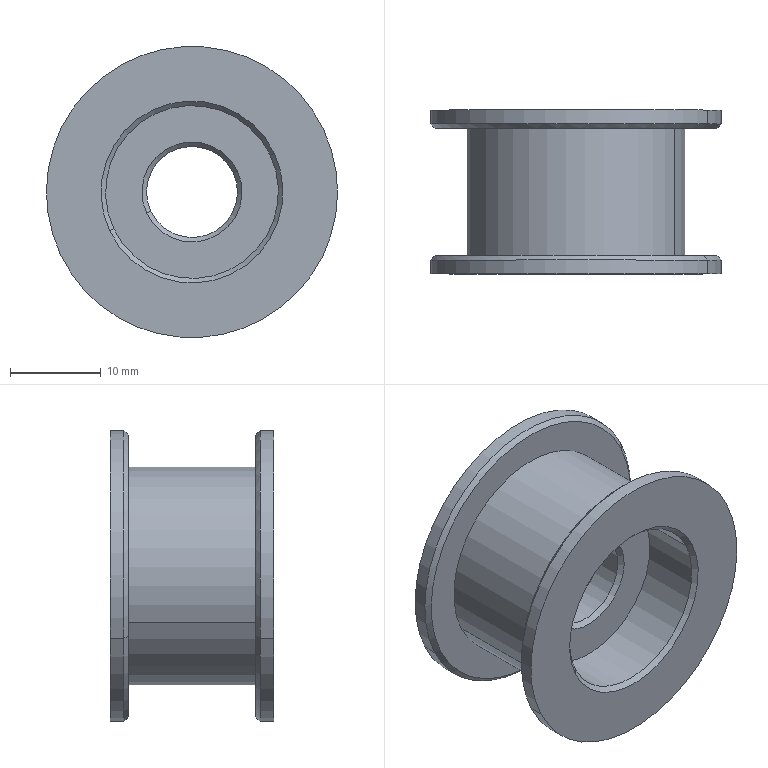Component | SolidWorks | Roller-1_BearingSleeve-1 | 1 solid | 30 faces | box 32 x 18 x 32 mm | volume 5219 mm3 | cone 12 | cylinder 12 | plane 6 | commonest cylinder face diameters 32 x4 19 x4 10 x2 24 x2
STEP:
#1=CARTESIAN_POINT('',(2.401,-2.146,10.487));
#2=VERTEX_POINT('',#1);
#3=CARTESIAN_POINT('',(3.505,-2.146,11.009));
#4=VERTEX_POINT('',#3);
#5=CARTESIAN_POINT('',(2.953,-2.146,10.748));
#6=DIRECTION('',(0.,1.,0.));
#7=DIRECTION('',(0.9043,0.,0.4269));
#8=AXIS2_PLACEMENT_3D('',#5,#6,#7);
#9=CIRCLE('',#8,0.6102);
#10=EDGE_CURVE('',#2,#4,#9,.T.);
#11=ORIENTED_EDGE('',*,*,#10,.F.);
#12=CARTESIAN_POINT('',(2.383,-2.165,10.479));
#13=VERTEX_POINT('',#12);
#14=CARTESIAN_POINT('',(2.383,-2.165,10.479));
#15=DIRECTION('',(-0.6394,-0.7071,-0.3019));
#16=VECTOR('',#15,39.37);
#17=LINE('',#14,#16);
#18=EDGE_CURVE('',#2,#13,#17,.T.);
#19=ORIENTED_EDGE('',*,*,#18,.T.);
#20=CARTESIAN_POINT('',(3.522,-2.165,11.017));
#21=VERTEX_POINT('',#20);
#22=CARTESIAN_POINT('',(2.953,-2.165,10.748));
#23=DIRECTION('',(0.,-1.,0.));
#24=DIRECTION('',(0.9043,0.,0.4269));
#25=AXIS2_PLACEMENT_3D('',#22,#23,#24);
#26=CIRCLE('',#25,0.6299);
#27=EDGE_CURVE('',#21,#13,#26,.T.);
#28=ORIENTED_EDGE('',*,*,#27,.F.);
#29=CARTESIAN_POINT('',(3.522,-2.165,11.017));
#30=DIRECTION('',(0.6394,-0.7071,0.3019));
#31=VECTOR('',#30,39.37);
#32=LINE('',#29,#31);
#33=EDGE_CURVE('',#4,#21,#32,.T.);
#34=ORIENTED_EDGE('',*,*,#33,.F.);
#35=EDGE_LOOP('',(#11,#19,#28,#34));
#36=FACE_OUTER_BOUND('',#35,.T.);
#37=CARTESIAN_POINT('',(2.953,-2.165,10.748));
#38=DIRECTION('',(0.,-1.,0.));
#39=DIRECTION('',(0.9043,0.,0.4269));
#40=AXIS2_PLACEMENT_3D('',#37,#38,#39);
#41=CONICAL_SURFACE('',#40,0.6299,0.7854);
#42=ADVANCED_FACE('',(#36),#41,.T.);
#43=CARTESIAN_POINT('',(3.505,-1.594,11.009));
#44=VERTEX_POINT('',#43);
#45=CARTESIAN_POINT('',(2.401,-1.594,10.487));
#46=VERTEX_POINT('',#45);
#47=CARTESIAN_POINT('',(2.953,-1.594,10.748));
#48=DIRECTION('',(0.,-1.,0.));
#49=DIRECTION('',(-0.9043,0.,-0.4269));
#50=AXIS2_PLACEMENT_3D('',#47,#48,#49);
#51=CIRCLE('',#50,0.6102);
#52=EDGE_CURVE('',#44,#46,#51,.T.);
#53=ORIENTED_EDGE('',*,*,#52,.F.);
#54=CARTESIAN_POINT('',(3.522,-1.575,11.017));
#55=VERTEX_POINT('',#54);
#56=CARTESIAN_POINT('',(3.522,-1.575,11.017));
#57=DIRECTION('',(0.6394,0.7071,0.3019));
#58=VECTOR('',#57,39.37);
#59=LINE('',#56,#58);
#60=EDGE_CURVE('',#44,#55,#59,.T.);
#61=ORIENTED_EDGE('',*,*,#60,.T.);
#62=CARTESIAN_POINT('',(2.383,-1.575,10.479));
#63=VERTEX_POINT('',#62);
#64=CARTESIAN_POINT('',(2.953,-1.575,10.748));
#65=DIRECTION('',(0.,1.,0.));
#66=DIRECTION('',(-0.9043,0.,-0.4269));
#67=AXIS2_PLACEMENT_3D('',#64,#65,#66);
#68=CIRCLE('',#67,0.6299);
#69=EDGE_CURVE('',#63,#55,#68,.T.);
#70=ORIENTED_EDGE('',*,*,#69,.F.);
#71=CARTESIAN_POINT('',(2.383,-1.575,10.479));
#72=DIRECTION('',(-0.6394,0.7071,-0.3019));
#73=VECTOR('',#72,39.37);
#74=LINE('',#71,#73);
#75=EDGE_CURVE('',#46,#63,#74,.T.);
#76=ORIENTED_EDGE('',*,*,#75,.F.);
#77=EDGE_LOOP('',(#53,#61,#70,#76));
#78=FACE_OUTER_BOUND('',#77,.T.);
#79=CARTESIAN_POINT('',(2.953,-1.575,10.748));
#80=DIRECTION('',(0.,1.,0.));
#81=DIRECTION('',(-0.9043,0.,-0.4269));
#82=AXIS2_PLACEMENT_3D('',#79,#80,#81);
#83=CONICAL_SURFACE('',#82,0.6299,0.7854);
#84=ADVANCED_FACE('',(#78),#83,.T.);
#85=CARTESIAN_POINT('',(2.615,-2.205,10.588));
#86=VERTEX_POINT('',#85);
#87=CARTESIAN_POINT('',(3.291,-2.205,10.908));
#88=VERTEX_POINT('',#87);
#89=CARTESIAN_POINT('',(2.953,-2.205,10.748));
#90=DIRECTION('',(0.,-1.,0.));
#91=DIRECTION('',(0.9043,0.,0.4269));
#92=AXIS2_PLACEMENT_3D('',#89,#90,#91);
#93=CIRCLE('',#92,0.374);
#94=EDGE_CURVE('',#86,#88,#93,.T.);
#95=ORIENTED_EDGE('',*,*,#94,.F.);
#96=CARTESIAN_POINT('',(2.597,-2.224,10.58));
#97=VERTEX_POINT('',#96);
#98=CARTESIAN_POINT('',(2.615,-2.205,10.588));
#99=DIRECTION('',(-0.6394,-0.7071,-0.3019));
#100=VECTOR('',#99,39.37);
#101=LINE('',#98,#100);
#102=EDGE_CURVE('',#86,#97,#101,.T.);
#103=ORIENTED_EDGE('',*,*,#102,.T.);
#104=CARTESIAN_POINT('',(3.309,-2.224,10.916));
#105=VERTEX_POINT('',#104);
#106=CARTESIAN_POINT('',(2.953,-2.224,10.748));
#107=DIRECTION('',(0.,1.,0.));
#108=DIRECTION('',(0.9043,0.,0.4269));
#109=AXIS2_PLACEMENT_3D('',#106,#107,#108);
#110=CIRCLE('',#109,0.3937);
#111=EDGE_CURVE('',#105,#97,#110,.T.);
#112=ORIENTED_EDGE('',*,*,#111,.F.);
#113=CARTESIAN_POINT('',(3.291,-2.205,10.908));
#114=DIRECTION('',(0.6394,-0.7071,0.3019));
#115=VECTOR('',#114,39.37);
#116=LINE('',#113,#115);
#117=EDGE_CURVE('',#88,#105,#116,.T.);
#118=ORIENTED_EDGE('',*,*,#117,.F.);
#119=EDGE_LOOP('',(#95,#103,#112,#118));
#120=FACE_OUTER_BOUND('',#119,.T.);
#121=CARTESIAN_POINT('',(2.953,-2.205,10.748));
#122=DIRECTION('',(0.,-1.,0.));
#123=DIRECTION('',(0.9043,0.,0.4269));
#124=AXIS2_PLACEMENT_3D('',#121,#122,#123);
#125=CONICAL_SURFACE('',#124,0.374,0.7854);
#126=ADVANCED_FACE('',(#120),#125,.F.);
#127=CARTESIAN_POINT('',(3.291,-1.535,10.908));
#128=VERTEX_POINT('',#127);
#129=CARTESIAN_POINT('',(2.615,-1.535,10.588));
#130=VERTEX_POINT('',#129);
#131=CARTESIAN_POINT('',(2.953,-1.535,10.748));
#132=DIRECTION('',(0.,1.,0.));
#133=DIRECTION('',(0.9043,0.,0.4269));
#134=AXIS2_PLACEMENT_3D('',#131,#132,#133);
#135=CIRCLE('',#134,0.374);
#136=EDGE_CURVE('',#128,#130,#135,.T.);
#137=ORIENTED_EDGE('',*,*,#136,.F.);
#138=CARTESIAN_POINT('',(3.309,-1.516,10.916));
#139=VERTEX_POINT('',#138);
#140=CARTESIAN_POINT('',(3.291,-1.535,10.908));
#141=DIRECTION('',(0.6394,0.7071,0.3019));
#142=VECTOR('',#141,39.37);
#143=LINE('',#140,#142);
#144=EDGE_CURVE('',#128,#139,#143,.T.);
#145=ORIENTED_EDGE('',*,*,#144,.T.);
#146=CARTESIAN_POINT('',(2.597,-1.516,10.58));
#147=VERTEX_POINT('',#146);
#148=CARTESIAN_POINT('',(2.953,-1.516,10.748));
#149=DIRECTION('',(0.,-1.,0.));
#150=DIRECTION('',(0.9043,0.,0.4269));
#151=AXIS2_PLACEMENT_3D('',#148,#149,#150);
#152=CIRCLE('',#151,0.3937);
#153=EDGE_CURVE('',#147,#139,#152,.T.);
#154=ORIENTED_EDGE('',*,*,#153,.F.);
#155=CARTESIAN_POINT('',(2.615,-1.535,10.588));
#156=DIRECTION('',(-0.6394,0.7071,-0.3019));
#157=VECTOR('',#156,39.37);
#158=LINE('',#155,#157);
#159=EDGE_CURVE('',#130,#147,#158,.T.);
#160=ORIENTED_EDGE('',*,*,#159,.F.);
#161=EDGE_LOOP('',(#137,#145,#154,#160));
#162=FACE_OUTER_BOUND('',#161,.T.);
#163=CARTESIAN_POINT('',(2.953,-1.535,10.748));
#164=DIRECTION('',(0.,1.,0.));
#165=DIRECTION('',(-0.9043,0.,-0.4269));
#166=AXIS2_PLACEMENT_3D('',#163,#164,#165);
#167=CONICAL_SURFACE('',#166,0.374,0.7854);
#168=ADVANCED_FACE('',(#162),#167,.F.);
#169=CARTESIAN_POINT('',(2.775,-1.929,10.664));
#170=VERTEX_POINT('',#169);
#171=CARTESIAN_POINT('',(3.131,-1.929,10.832));
#172=VERTEX_POINT('',#171);
#173=CARTESIAN_POINT('',(2.953,-1.929,10.748));
#174=DIRECTION('',(0.,-1.,0.));
#175=DIRECTION('',(0.9043,0.,0.4269));
#176=AXIS2_PLACEMENT_3D('',#173,#174,#175);
#177=CIRCLE('',#176,0.1969);
#178=EDGE_CURVE('',#170,#172,#177,.T.);
#179=ORIENTED_EDGE('',*,*,#178,.F.);
#180=CARTESIAN_POINT('',(2.757,-1.949,10.656));
#181=VERTEX_POINT('',#180);
#182=CARTESIAN_POINT('',(2.775,-1.929,10.664));
#183=DIRECTION('',(-0.6394,-0.7071,-0.3019));
#184=VECTOR('',#183,39.37);
#185=LINE('',#182,#184);
#186=EDGE_CURVE('',#170,#181,#185,.T.);
#187=ORIENTED_EDGE('',*,*,#186,.T.);
#188=CARTESIAN_POINT('',(3.149,-1.949,10.84));
#189=VERTEX_POINT('',#188);
#190=CARTESIAN_POINT('',(2.953,-1.949,10.748));
#191=DIRECTION('',(0.,1.,0.));
#192=DIRECTION('',(0.9043,0.,0.4269));
#193=AXIS2_PLACEMENT_3D('',#190,#191,#192);
#194=CIRCLE('',#193,0.2165);
#195=EDGE_CURVE('',#189,#181,#194,.T.);
#196=ORIENTED_EDGE('',*,*,#195,.F.);
#197=CARTESIAN_POINT('',(3.131,-1.929,10.832));
#198=DIRECTION('',(0.6394,-0.7071,0.3019));
#199=VECTOR('',#198,39.37);
#200=LINE('',#197,#199);
#201=EDGE_CURVE('',#172,#189,#200,.T.);
#202=ORIENTED_EDGE('',*,*,#201,.F.);
#203=EDGE_LOOP('',(#179,#187,#196,#202));
#204=FACE_OUTER_BOUND('',#203,.T.);
#205=CARTESIAN_POINT('',(2.953,-1.929,10.748));
#206=DIRECTION('',(0.,-1.,0.));
#207=DIRECTION('',(0.9043,0.,0.4269));
#208=AXIS2_PLACEMENT_3D('',#205,#206,#207);
#209=CONICAL_SURFACE('',#208,0.1969,0.7854);
#210=ADVANCED_FACE('',(#204),#209,.F.);
#211=CARTESIAN_POINT('',(3.131,-1.811,10.832));
#212=VERTEX_POINT('',#211);
#213=CARTESIAN_POINT('',(2.775,-1.811,10.664));
#214=VERTEX_POINT('',#213);
#215=CARTESIAN_POINT('',(2.953,-1.811,10.748));
#216=DIRECTION('',(0.,1.,0.));
#217=DIRECTION('',(-0.9043,0.,-0.4269));
#218=AXIS2_PLACEMENT_3D('',#215,#216,#217);
#219=CIRCLE('',#218,0.1969);
#220=EDGE_CURVE('',#212,#214,#219,.T.);
#221=ORIENTED_EDGE('',*,*,#220,.F.);
#222=CARTESIAN_POINT('',(3.149,-1.791,10.84));
#223=VERTEX_POINT('',#222);
#224=CARTESIAN_POINT('',(3.131,-1.811,10.832));
#225=DIRECTION('',(0.6394,0.7071,0.3019));
#226=VECTOR('',#225,39.37);
#227=LINE('',#224,#226);
#228=EDGE_CURVE('',#212,#223,#227,.T.);
#229=ORIENTED_EDGE('',*,*,#228,.T.);
#230=CARTESIAN_POINT('',(2.757,-1.791,10.656));
#231=VERTEX_POINT('',#230);
#232=CARTESIAN_POINT('',(2.953,-1.791,10.748));
#233=DIRECTION('',(0.,-1.,0.));
#234=DIRECTION('',(-0.9043,0.,-0.4269));
#235=AXIS2_PLACEMENT_3D('',#232,#233,#234);
#236=CIRCLE('',#235,0.2165);
#237=EDGE_CURVE('',#231,#223,#236,.T.);
#238=ORIENTED_EDGE('',*,*,#237,.F.);
#239=CARTESIAN_POINT('',(2.775,-1.811,10.664));
#240=DIRECTION('',(-0.6394,0.7071,-0.3019));
#241=VECTOR('',#240,39.37);
#242=LINE('',#239,#241);
#243=EDGE_CURVE('',#214,#231,#242,.T.);
#244=ORIENTED_EDGE('',*,*,#243,.F.);
#245=EDGE_LOOP('',(#221,#229,#238,#244));
#246=FACE_OUTER_BOUND('',#245,.T.);
#247=CARTESIAN_POINT('',(2.953,-1.811,10.748));
#248=DIRECTION('',(0.,1.,0.));
#249=DIRECTION('',(-0.9043,0.,-0.4269));
#250=AXIS2_PLACEMENT_3D('',#247,#248,#249);
#251=CONICAL_SURFACE('',#250,0.1969,0.7854);
#252=ADVANCED_FACE('',(#246),#251,.F.);
#253=ORIENTED_EDGE('',*,*,#69,.T.);
#254=CARTESIAN_POINT('',(3.522,-1.516,11.017));
#255=VERTEX_POINT('',#254);
#256=CARTESIAN_POINT('',(3.522,-1.594,11.017));
#257=DIRECTION('',(0.,1.,0.));
#258=VECTOR('',#257,39.37);
#259=LINE('',#256,#258);
#260=EDGE_CURVE('',#55,#255,#259,.T.);
#261=ORIENTED_EDGE('',*,*,#260,.T.);
#262=CARTESIAN_POINT('',(2.383,-1.516,10.479));
#263=VERTEX_POINT('',#262);
#264=CARTESIAN_POINT('',(2.953,-1.516,10.748));
#265=DIRECTION('',(0.,1.,0.));
#266=DIRECTION('',(-0.9043,0.,-0.4269));
#267=AXIS2_PLACEMENT_3D('',#264,#265,#266);
#268=CIRCLE('',#267,0.6299);
#269=EDGE_CURVE('',#263,#255,#268,.T.);
#270=ORIENTED_EDGE('',*,*,#269,.F.);
#271=CARTESIAN_POINT('',(2.383,-1.594,10.479));
#272=DIRECTION('',(0.,1.,0.));
#273=VECTOR('',#272,39.37);
#274=LINE('',#271,#273);
#275=EDGE_CURVE('',#63,#263,#274,.T.);
#276=ORIENTED_EDGE('',*,*,#275,.F.);
#277=EDGE_LOOP('',(#253,#261,#270,#276));
#278=FACE_OUTER_BOUND('',#277,.T.);
#279=CARTESIAN_POINT('',(2.953,-1.594,10.748));
#280=DIRECTION('',(0.,1.,0.));
#281=DIRECTION('',(-0.9043,0.,-0.4269));
#282=AXIS2_PLACEMENT_3D('',#279,#280,#281);
#283=CYLINDRICAL_SURFACE('',#282,0.6299);
#284=ADVANCED_FACE('',(#278),#283,.T.);
#285=ORIENTED_EDGE('',*,*,#27,.T.);
#286=CARTESIAN_POINT('',(2.383,-2.224,10.479));
#287=VERTEX_POINT('',#286);
#288=CARTESIAN_POINT('',(2.383,-2.146,10.479));
#289=DIRECTION('',(0.,-1.,0.));
#290=VECTOR('',#289,39.37);
#291=LINE('',#288,#290);
#292=EDGE_CURVE('',#13,#287,#291,.T.);
#293=ORIENTED_EDGE('',*,*,#292,.T.);
#294=CARTESIAN_POINT('',(3.522,-2.224,11.017));
#295=VERTEX_POINT('',#294);
#296=CARTESIAN_POINT('',(2.953,-2.224,10.748));
#297=DIRECTION('',(0.,-1.,0.));
#298=DIRECTION('',(0.9043,0.,0.4269));
#299=AXIS2_PLACEMENT_3D('',#296,#297,#298);
#300=CIRCLE('',#299,0.6299);
#301=EDGE_CURVE('',#295,#287,#300,.T.);
#302=ORIENTED_EDGE('',*,*,#301,.F.);
#303=CARTESIAN_POINT('',(3.522,-2.146,11.017));
#304=DIRECTION('',(0.,-1.,0.));
#305=VECTOR('',#304,39.37);
#306=LINE('',#303,#305);
#307=EDGE_CURVE('',#21,#295,#306,.T.);
#308=ORIENTED_EDGE('',*,*,#307,.F.);
#309=EDGE_LOOP('',(#285,#293,#302,#308));
#310=FACE_OUTER_BOUND('',#309,.T.);
#311=CARTESIAN_POINT('',(2.953,-2.146,10.748));
#312=DIRECTION('',(0.,-1.,0.));
#313=DIRECTION('',(0.9043,0.,0.4269));
#314=AXIS2_PLACEMENT_3D('',#311,#312,#313);
#315=CYLINDRICAL_SURFACE('',#314,0.6299);
#316=ADVANCED_FACE('',(#310),#315,.T.);
#317=ORIENTED_EDGE('',*,*,#178,.T.);
#318=CARTESIAN_POINT('',(3.131,-2.067,10.832));
#319=DIRECTION('',(0.,1.,0.));
#320=VECTOR('',#319,39.37);
#321=LINE('',#318,#320);
#322=EDGE_CURVE('',#172,#212,#321,.T.);
#323=ORIENTED_EDGE('',*,*,#322,.T.);
#324=ORIENTED_EDGE('',*,*,#220,.T.);
#325=CARTESIAN_POINT('',(2.775,-2.067,10.664));
#326=DIRECTION('',(0.,1.,0.));
#327=VECTOR('',#326,39.37);
#328=LINE('',#325,#327);
#329=EDGE_CURVE('',#170,#214,#328,.T.);
#330=ORIENTED_EDGE('',*,*,#329,.F.);
#331=EDGE_LOOP('',(#317,#323,#324,#330));
#332=FACE_OUTER_BOUND('',#331,.T.);
#333=CARTESIAN_POINT('',(2.953,-2.067,10.748));
#334=DIRECTION('',(0.,1.,0.));
#335=DIRECTION('',(-0.9043,0.,-0.4269));
#336=AXIS2_PLACEMENT_3D('',#333,#334,#335);
#337=CYLINDRICAL_SURFACE('',#336,0.1969);
#338=ADVANCED_FACE('',(#332),#337,.F.);
#339=CARTESIAN_POINT('',(3.291,-1.791,10.908));
#340=VERTEX_POINT('',#339);
#341=CARTESIAN_POINT('',(2.615,-1.791,10.588));
#342=VERTEX_POINT('',#341);
#343=CARTESIAN_POINT('',(2.953,-1.791,10.748));
#344=DIRECTION('',(0.,1.,0.));
#345=DIRECTION('',(-0.9043,0.,-0.4269));
#346=AXIS2_PLACEMENT_3D('',#343,#344,#345);
#347=CIRCLE('',#346,0.374);
#348=EDGE_CURVE('',#340,#342,#347,.T.);
#349=ORIENTED_EDGE('',*,*,#348,.F.);
#350=CARTESIAN_POINT('',(3.291,-1.791,10.908));
#351=DIRECTION('',(0.,1.,0.));
#352=VECTOR('',#351,39.37);
#353=LINE('',#350,#352);
#354=EDGE_CURVE('',#340,#128,#353,.T.);
#355=ORIENTED_EDGE('',*,*,#354,.T.);
#356=ORIENTED_EDGE('',*,*,#136,.T.);
#357=CARTESIAN_POINT('',(2.615,-1.791,10.588));
#358=DIRECTION('',(0.,1.,0.));
#359=VECTOR('',#358,39.37);
#360=LINE('',#357,#359);
#361=EDGE_CURVE('',#342,#130,#360,.T.);
#362=ORIENTED_EDGE('',*,*,#361,.F.);
#363=EDGE_LOOP('',(#349,#355,#356,#362));
#364=FACE_OUTER_BOUND('',#363,.T.);
#365=CARTESIAN_POINT('',(2.953,-1.791,10.748));
#366=DIRECTION('',(0.,1.,0.));
#367=DIRECTION('',(-0.9043,0.,-0.4269));
#368=AXIS2_PLACEMENT_3D('',#365,#366,#367);
#369=CYLINDRICAL_SURFACE('',#368,0.374);
#370=ADVANCED_FACE('',(#364),#369,.F.);
#371=CARTESIAN_POINT('',(2.615,-1.949,10.588));
#372=VERTEX_POINT('',#371);
#373=CARTESIAN_POINT('',(3.291,-1.949,10.908));
#374=VERTEX_POINT('',#373);
#375=CARTESIAN_POINT('',(2.953,-1.949,10.748));
#376=DIRECTION('',(0.,-1.,0.));
#377=DIRECTION('',(0.9043,0.,0.4269));
#378=AXIS2_PLACEMENT_3D('',#375,#376,#377);
#379=CIRCLE('',#378,0.374);
#380=EDGE_CURVE('',#372,#374,#379,.T.);
#381=ORIENTED_EDGE('',*,*,#380,.F.);
#382=CARTESIAN_POINT('',(2.615,-1.949,10.588));
#383=DIRECTION('',(0.,-1.,0.));
#384=VECTOR('',#383,39.37);
#385=LINE('',#382,#384);
#386=EDGE_CURVE('',#372,#86,#385,.T.);
#387=ORIENTED_EDGE('',*,*,#386,.T.);
#388=ORIENTED_EDGE('',*,*,#94,.T.);
#389=CARTESIAN_POINT('',(3.291,-1.949,10.908));
#390=DIRECTION('',(0.,-1.,0.));
#391=VECTOR('',#390,39.37);
#392=LINE('',#389,#391);
#393=EDGE_CURVE('',#374,#88,#392,.T.);
#394=ORIENTED_EDGE('',*,*,#393,.F.);
#395=EDGE_LOOP('',(#381,#387,#388,#394));
#396=FACE_OUTER_BOUND('',#395,.T.);
#397=CARTESIAN_POINT('',(2.953,-1.949,10.748));
#398=DIRECTION('',(0.,-1.,0.));
#399=DIRECTION('',(0.9043,0.,0.4269));
#400=AXIS2_PLACEMENT_3D('',#397,#398,#399);
#401=CYLINDRICAL_SURFACE('',#400,0.374);
#402=ADVANCED_FACE('',(#396),#401,.F.);
#403=CARTESIAN_POINT('',(3.38,-2.146,10.95));
#404=VERTEX_POINT('',#403);
#405=CARTESIAN_POINT('',(2.526,-2.146,10.546));
#406=VERTEX_POINT('',#405);
#407=CARTESIAN_POINT('',(2.953,-2.146,10.748));
#408=DIRECTION('',(0.,-1.,0.));
#409=DIRECTION('',(0.9043,0.,0.4269));
#410=AXIS2_PLACEMENT_3D('',#407,#408,#409);
#411=CIRCLE('',#410,0.4724);
#412=EDGE_CURVE('',#404,#406,#411,.T.);
#413=ORIENTED_EDGE('',*,*,#412,.F.);
#414=CARTESIAN_POINT('',(3.38,-1.594,10.95));
#415=VERTEX_POINT('',#414);
#416=CARTESIAN_POINT('',(3.38,-2.224,10.95));
#417=DIRECTION('',(0.,1.,0.));
#418=VECTOR('',#417,39.37);
#419=LINE('',#416,#418);
#420=EDGE_CURVE('',#404,#415,#419,.T.);
#421=ORIENTED_EDGE('',*,*,#420,.T.);
#422=CARTESIAN_POINT('',(2.526,-1.594,10.546));
#423=VERTEX_POINT('',#422);
#424=CARTESIAN_POINT('',(2.953,-1.594,10.748));
#425=DIRECTION('',(0.,1.,0.));
#426=DIRECTION('',(-0.9043,0.,-0.4269));
#427=AXIS2_PLACEMENT_3D('',#424,#425,#426);
#428=CIRCLE('',#427,0.4724);
#429=EDGE_CURVE('',#423,#415,#428,.T.);
#430=ORIENTED_EDGE('',*,*,#429,.F.);
#431=CARTESIAN_POINT('',(2.526,-2.224,10.546));
#432=DIRECTION('',(0.,1.,0.));
#433=VECTOR('',#432,39.37);
#434=LINE('',#431,#433);
#435=EDGE_CURVE('',#406,#423,#434,.T.);
#436=ORIENTED_EDGE('',*,*,#435,.F.);
#437=EDGE_LOOP('',(#413,#421,#430,#436));
#438=FACE_OUTER_BOUND('',#437,.T.);
#439=CARTESIAN_POINT('',(2.953,-2.224,10.748));
#440=DIRECTION('',(0.,1.,0.));
#441=DIRECTION('',(-0.9043,0.,-0.4269));
#442=AXIS2_PLACEMENT_3D('',#439,#440,#441);
#443=CYLINDRICAL_SURFACE('',#442,0.4724);
#444=ADVANCED_FACE('',(#438),#443,.T.);
#445=ORIENTED_EDGE('',*,*,#429,.T.);
#446=CARTESIAN_POINT('',(2.953,-1.594,10.748));
#447=DIRECTION('',(0.,1.,0.));
#448=DIRECTION('',(-0.9043,0.,-0.4269));
#449=AXIS2_PLACEMENT_3D('',#446,#447,#448);
#450=CIRCLE('',#449,0.4724);
#451=EDGE_CURVE('',#415,#423,#450,.T.);
#452=ORIENTED_EDGE('',*,*,#451,.T.);
#453=EDGE_LOOP('',(#445,#452));
#454=FACE_BOUND('',#453,.T.);
#455=CARTESIAN_POINT('',(2.953,-1.594,10.748));
#456=DIRECTION('',(0.,-1.,0.));
#457=DIRECTION('',(-0.9043,0.,-0.4269));
#458=AXIS2_PLACEMENT_3D('',#455,#456,#457);
#459=CIRCLE('',#458,0.6102);
#460=EDGE_CURVE('',#46,#44,#459,.T.);
#461=ORIENTED_EDGE('',*,*,#460,.T.);
#462=ORIENTED_EDGE('',*,*,#52,.T.);
#463=EDGE_LOOP('',(#461,#462));
#464=FACE_OUTER_BOUND('',#463,.T.);
#465=CARTESIAN_POINT('',(2.953,-1.594,10.748));
#466=DIRECTION('',(0.,1.,0.));
#467=DIRECTION('',(0.4269,0.,-0.9043));
#468=AXIS2_PLACEMENT_3D('',#465,#466,#467);
#469=PLANE('',#468);
#470=ADVANCED_FACE('',(#454,#464),#469,.F.);
#471=CARTESIAN_POINT('',(2.953,-2.146,10.748));
#472=DIRECTION('',(0.,-1.,0.));
#473=DIRECTION('',(0.9043,0.,0.4269));
#474=AXIS2_PLACEMENT_3D('',#471,#472,#473);
#475=CIRCLE('',#474,0.4724);
#476=EDGE_CURVE('',#406,#404,#475,.T.);
#477=ORIENTED_EDGE('',*,*,#476,.T.);
#478=ORIENTED_EDGE('',*,*,#412,.T.);
#479=EDGE_LOOP('',(#477,#478));
#480=FACE_BOUND('',#479,.T.);
#481=CARTESIAN_POINT('',(2.953,-2.146,10.748));
#482=DIRECTION('',(0.,1.,0.));
#483=DIRECTION('',(0.9043,0.,0.4269));
#484=AXIS2_PLACEMENT_3D('',#481,#482,#483);
#485=CIRCLE('',#484,0.6102);
#486=EDGE_CURVE('',#4,#2,#485,.T.);
#487=ORIENTED_EDGE('',*,*,#486,.T.);
#488=ORIENTED_EDGE('',*,*,#10,.T.);
#489=EDGE_LOOP('',(#487,#488));
#490=FACE_OUTER_BOUND('',#489,.T.);
#491=CARTESIAN_POINT('',(2.953,-2.146,10.748));
#492=DIRECTION('',(0.,-1.,0.));
#493=DIRECTION('',(0.9043,0.,0.4269));
#494=AXIS2_PLACEMENT_3D('',#491,#492,#493);
#495=PLANE('',#494);
#496=ADVANCED_FACE('',(#480,#490),#495,.F.);
#497=ORIENTED_EDGE('',*,*,#237,.T.);
#498=CARTESIAN_POINT('',(2.953,-1.791,10.748));
#499=DIRECTION('',(0.,-1.,0.));
#500=DIRECTION('',(-0.9043,0.,-0.4269));
#501=AXIS2_PLACEMENT_3D('',#498,#499,#500);
#502=CIRCLE('',#501,0.2165);
#503=EDGE_CURVE('',#223,#231,#502,.T.);
#504=ORIENTED_EDGE('',*,*,#503,.T.);
#505=EDGE_LOOP('',(#497,#504));
#506=FACE_BOUND('',#505,.T.);
#507=CARTESIAN_POINT('',(2.953,-1.791,10.748));
#508=DIRECTION('',(0.,1.,0.));
#509=DIRECTION('',(-0.9043,0.,-0.4269));
#510=AXIS2_PLACEMENT_3D('',#507,#508,#509);
#511=CIRCLE('',#510,0.374);
#512=EDGE_CURVE('',#342,#340,#511,.T.);
#513=ORIENTED_EDGE('',*,*,#512,.T.);
#514=ORIENTED_EDGE('',*,*,#348,.T.);
#515=EDGE_LOOP('',(#513,#514));
#516=FACE_OUTER_BOUND('',#515,.T.);
#517=CARTESIAN_POINT('',(2.953,-1.791,10.748));
#518=DIRECTION('',(0.,1.,0.));
#519=DIRECTION('',(0.4269,0.,-0.9043));
#520=AXIS2_PLACEMENT_3D('',#517,#518,#519);
#521=PLANE('',#520);
#522=ADVANCED_FACE('',(#506,#516),#521,.T.);
#523=ORIENTED_EDGE('',*,*,#195,.T.);
#524=CARTESIAN_POINT('',(2.953,-1.949,10.748));
#525=DIRECTION('',(0.,1.,0.));
#526=DIRECTION('',(0.9043,0.,0.4269));
#527=AXIS2_PLACEMENT_3D('',#524,#525,#526);
#528=CIRCLE('',#527,0.2165);
#529=EDGE_CURVE('',#181,#189,#528,.T.);
#530=ORIENTED_EDGE('',*,*,#529,.T.);
#531=EDGE_LOOP('',(#523,#530));
#532=FACE_BOUND('',#531,.T.);
#533=CARTESIAN_POINT('',(2.953,-1.949,10.748));
#534=DIRECTION('',(0.,-1.,0.));
#535=DIRECTION('',(0.9043,0.,0.4269));
#536=AXIS2_PLACEMENT_3D('',#533,#534,#535);
#537=CIRCLE('',#536,0.374);
#538=EDGE_CURVE('',#374,#372,#537,.T.);
#539=ORIENTED_EDGE('',*,*,#538,.T.);
#540=ORIENTED_EDGE('',*,*,#380,.T.);
#541=EDGE_LOOP('',(#539,#540));
#542=FACE_OUTER_BOUND('',#541,.T.);
#543=CARTESIAN_POINT('',(2.953,-1.949,10.748));
#544=DIRECTION('',(0.,-1.,0.));
#545=DIRECTION('',(0.9043,0.,0.4269));
#546=AXIS2_PLACEMENT_3D('',#543,#544,#545);
#547=PLANE('',#546);
#548=ADVANCED_FACE('',(#532,#542),#547,.T.);
#549=ORIENTED_EDGE('',*,*,#153,.T.);
#550=CARTESIAN_POINT('',(2.953,-1.516,10.748));
#551=DIRECTION('',(0.,-1.,0.));
#552=DIRECTION('',(0.9043,0.,0.4269));
#553=AXIS2_PLACEMENT_3D('',#550,#551,#552);
#554=CIRCLE('',#553,0.3937);
#555=EDGE_CURVE('',#139,#147,#554,.T.);
#556=ORIENTED_EDGE('',*,*,#555,.T.);
#557=EDGE_LOOP('',(#549,#556));
#558=FACE_BOUND('',#557,.T.);
#559=ORIENTED_EDGE('',*,*,#269,.T.);
#560=CARTESIAN_POINT('',(2.953,-1.516,10.748));
#561=DIRECTION('',(0.,1.,0.));
#562=DIRECTION('',(-0.9043,0.,-0.4269));
#563=AXIS2_PLACEMENT_3D('',#560,#561,#562);
#564=CIRCLE('',#563,0.6299);
#565=EDGE_CURVE('',#255,#263,#564,.T.);
#566=ORIENTED_EDGE('',*,*,#565,.T.);
#567=EDGE_LOOP('',(#559,#566));
#568=FACE_OUTER_BOUND('',#567,.T.);
#569=CARTESIAN_POINT('',(2.953,-1.516,10.748));
#570=DIRECTION('',(0.,-1.,0.));
#571=DIRECTION('',(0.9043,0.,0.4269));
#572=AXIS2_PLACEMENT_3D('',#569,#570,#571);
#573=PLANE('',#572);
#574=ADVANCED_FACE('',(#558,#568),#573,.F.);
#575=ORIENTED_EDGE('',*,*,#111,.T.);
#576=CARTESIAN_POINT('',(2.953,-2.224,10.748));
#577=DIRECTION('',(0.,1.,0.));
#578=DIRECTION('',(0.9043,0.,0.4269));
#579=AXIS2_PLACEMENT_3D('',#576,#577,#578);
#580=CIRCLE('',#579,0.3937);
#581=EDGE_CURVE('',#97,#105,#580,.T.);
#582=ORIENTED_EDGE('',*,*,#581,.T.);
#583=EDGE_LOOP('',(#575,#582));
#584=FACE_BOUND('',#583,.T.);
#585=ORIENTED_EDGE('',*,*,#301,.T.);
#586=CARTESIAN_POINT('',(2.953,-2.224,10.748));
#587=DIRECTION('',(0.,-1.,0.));
#588=DIRECTION('',(0.9043,0.,0.4269));
#589=AXIS2_PLACEMENT_3D('',#586,#587,#588);
#590=CIRCLE('',#589,0.6299);
#591=EDGE_CURVE('',#287,#295,#590,.T.);
#592=ORIENTED_EDGE('',*,*,#591,.T.);
#593=EDGE_LOOP('',(#585,#592));
#594=FACE_OUTER_BOUND('',#593,.T.);
#595=CARTESIAN_POINT('',(2.953,-2.224,10.748));
#596=DIRECTION('',(0.,-1.,0.));
#597=DIRECTION('',(0.9043,0.,0.4269));
#598=AXIS2_PLACEMENT_3D('',#595,#596,#597);
#599=PLANE('',#598);
#600=ADVANCED_FACE('',(#584,#594),#599,.T.);
#601=ORIENTED_EDGE('',*,*,#420,.F.);
#602=ORIENTED_EDGE('',*,*,#476,.F.);
#603=ORIENTED_EDGE('',*,*,#435,.T.);
#604=ORIENTED_EDGE('',*,*,#451,.F.);
#605=EDGE_LOOP('',(#601,#602,#603,#604));
#606=FACE_OUTER_BOUND('',#605,.T.);
#607=CARTESIAN_POINT('',(2.953,-2.224,10.748));
#608=DIRECTION('',(0.,1.,0.));
#609=DIRECTION('',(-0.9043,0.,-0.4269));
#610=AXIS2_PLACEMENT_3D('',#607,#608,#609);
#611=CYLINDRICAL_SURFACE('',#610,0.4724);
#612=ADVANCED_FACE('',(#606),#611,.T.);
#613=ORIENTED_EDGE('',*,*,#386,.F.);
#614=ORIENTED_EDGE('',*,*,#538,.F.);
#615=ORIENTED_EDGE('',*,*,#393,.T.);
#616=CARTESIAN_POINT('',(2.953,-2.205,10.748));
#617=DIRECTION('',(0.,-1.,0.));
#618=DIRECTION('',(0.9043,0.,0.4269));
#619=AXIS2_PLACEMENT_3D('',#616,#617,#618);
#620=CIRCLE('',#619,0.374);
#621=EDGE_CURVE('',#88,#86,#620,.T.);
#622=ORIENTED_EDGE('',*,*,#621,.T.);
#623=EDGE_LOOP('',(#613,#614,#615,#622));
#624=FACE_OUTER_BOUND('',#623,.T.);
#625=CARTESIAN_POINT('',(2.953,-1.949,10.748));
#626=DIRECTION('',(0.,-1.,0.));
#627=DIRECTION('',(0.9043,0.,0.4269));
#628=AXIS2_PLACEMENT_3D('',#625,#626,#627);
#629=CYLINDRICAL_SURFACE('',#628,0.374);
#630=ADVANCED_FACE('',(#624),#629,.F.);
#631=ORIENTED_EDGE('',*,*,#354,.F.);
#632=ORIENTED_EDGE('',*,*,#512,.F.);
#633=ORIENTED_EDGE('',*,*,#361,.T.);
#634=CARTESIAN_POINT('',(2.953,-1.535,10.748));
#635=DIRECTION('',(0.,1.,0.));
#636=DIRECTION('',(0.9043,0.,0.4269));
#637=AXIS2_PLACEMENT_3D('',#634,#635,#636);
#638=CIRCLE('',#637,0.374);
#639=EDGE_CURVE('',#130,#128,#638,.T.);
#640=ORIENTED_EDGE('',*,*,#639,.T.);
#641=EDGE_LOOP('',(#631,#632,#633,#640));
#642=FACE_OUTER_BOUND('',#641,.T.);
#643=CARTESIAN_POINT('',(2.953,-1.791,10.748));
#644=DIRECTION('',(0.,1.,0.));
#645=DIRECTION('',(-0.9043,0.,-0.4269));
#646=AXIS2_PLACEMENT_3D('',#643,#644,#645);
#647=CYLINDRICAL_SURFACE('',#646,0.374);
#648=ADVANCED_FACE('',(#642),#647,.F.);
#649=ORIENTED_EDGE('',*,*,#322,.F.);
#650=CARTESIAN_POINT('',(2.953,-1.929,10.748));
#651=DIRECTION('',(0.,-1.,0.));
#652=DIRECTION('',(0.9043,0.,0.4269));
#653=AXIS2_PLACEMENT_3D('',#650,#651,#652);
#654=CIRCLE('',#653,0.1969);
#655=EDGE_CURVE('',#172,#170,#654,.T.);
#656=ORIENTED_EDGE('',*,*,#655,.T.);
#657=ORIENTED_EDGE('',*,*,#329,.T.);
#658=CARTESIAN_POINT('',(2.953,-1.811,10.748));
#659=DIRECTION('',(0.,1.,0.));
#660=DIRECTION('',(-0.9043,0.,-0.4269));
#661=AXIS2_PLACEMENT_3D('',#658,#659,#660);
#662=CIRCLE('',#661,0.1969);
#663=EDGE_CURVE('',#214,#212,#662,.T.);
#664=ORIENTED_EDGE('',*,*,#663,.T.);
#665=EDGE_LOOP('',(#649,#656,#657,#664));
#666=FACE_OUTER_BOUND('',#665,.T.);
#667=CARTESIAN_POINT('',(2.953,-2.067,10.748));
#668=DIRECTION('',(0.,1.,0.));
#669=DIRECTION('',(-0.9043,0.,-0.4269));
#670=AXIS2_PLACEMENT_3D('',#667,#668,#669);
#671=CYLINDRICAL_SURFACE('',#670,0.1969);
#672=ADVANCED_FACE('',(#666),#671,.F.);
#673=ORIENTED_EDGE('',*,*,#292,.F.);
#674=CARTESIAN_POINT('',(2.953,-2.165,10.748));
#675=DIRECTION('',(0.,-1.,0.));
#676=DIRECTION('',(0.9043,0.,0.4269));
#677=AXIS2_PLACEMENT_3D('',#674,#675,#676);
#678=CIRCLE('',#677,0.6299);
#679=EDGE_CURVE('',#13,#21,#678,.T.);
#680=ORIENTED_EDGE('',*,*,#679,.T.);
#681=ORIENTED_EDGE('',*,*,#307,.T.);
#682=ORIENTED_EDGE('',*,*,#591,.F.);
#683=EDGE_LOOP('',(#673,#680,#681,#682));
#684=FACE_OUTER_BOUND('',#683,.T.);
#685=CARTESIAN_POINT('',(2.953,-2.146,10.748));
#686=DIRECTION('',(0.,-1.,0.));
#687=DIRECTION('',(0.9043,0.,0.4269));
#688=AXIS2_PLACEMENT_3D('',#685,#686,#687);
#689=CYLINDRICAL_SURFACE('',#688,0.6299);
#690=ADVANCED_FACE('',(#684),#689,.T.);
#691=ORIENTED_EDGE('',*,*,#260,.F.);
#692=CARTESIAN_POINT('',(2.953,-1.575,10.748));
#693=DIRECTION('',(0.,1.,0.));
#694=DIRECTION('',(-0.9043,0.,-0.4269));
#695=AXIS2_PLACEMENT_3D('',#692,#693,#694);
#696=CIRCLE('',#695,0.6299);
#697=EDGE_CURVE('',#55,#63,#696,.T.);
#698=ORIENTED_EDGE('',*,*,#697,.T.);
#699=ORIENTED_EDGE('',*,*,#275,.T.);
#700=ORIENTED_EDGE('',*,*,#565,.F.);
#701=EDGE_LOOP('',(#691,#698,#699,#700));
#702=FACE_OUTER_BOUND('',#701,.T.);
#703=CARTESIAN_POINT('',(2.953,-1.594,10.748));
#704=DIRECTION('',(0.,1.,0.));
#705=DIRECTION('',(-0.9043,0.,-0.4269));
#706=AXIS2_PLACEMENT_3D('',#703,#704,#705);
#707=CYLINDRICAL_SURFACE('',#706,0.6299);
#708=ADVANCED_FACE('',(#702),#707,.T.);
#709=ORIENTED_EDGE('',*,*,#228,.F.);
#710=ORIENTED_EDGE('',*,*,#663,.F.);
#711=ORIENTED_EDGE('',*,*,#243,.T.);
#712=ORIENTED_EDGE('',*,*,#503,.F.);
#713=EDGE_LOOP('',(#709,#710,#711,#712));
#714=FACE_OUTER_BOUND('',#713,.T.);
#715=CARTESIAN_POINT('',(2.953,-1.811,10.748));
#716=DIRECTION('',(0.,1.,0.));
#717=DIRECTION('',(-0.9043,0.,-0.4269));
#718=AXIS2_PLACEMENT_3D('',#715,#716,#717);
#719=CONICAL_SURFACE('',#718,0.1969,0.7854);
#720=ADVANCED_FACE('',(#714),#719,.F.);
#721=ORIENTED_EDGE('',*,*,#186,.F.);
#722=ORIENTED_EDGE('',*,*,#655,.F.);
#723=ORIENTED_EDGE('',*,*,#201,.T.);
#724=ORIENTED_EDGE('',*,*,#529,.F.);
#725=EDGE_LOOP('',(#721,#722,#723,#724));
#726=FACE_OUTER_BOUND('',#725,.T.);
#727=CARTESIAN_POINT('',(2.953,-1.929,10.748));
#728=DIRECTION('',(0.,-1.,0.));
#729=DIRECTION('',(0.9043,0.,0.4269));
#730=AXIS2_PLACEMENT_3D('',#727,#728,#729);
#731=CONICAL_SURFACE('',#730,0.1969,0.7854);
#732=ADVANCED_FACE('',(#726),#731,.F.);
#733=ORIENTED_EDGE('',*,*,#144,.F.);
#734=ORIENTED_EDGE('',*,*,#639,.F.);
#735=ORIENTED_EDGE('',*,*,#159,.T.);
#736=ORIENTED_EDGE('',*,*,#555,.F.);
#737=EDGE_LOOP('',(#733,#734,#735,#736));
#738=FACE_OUTER_BOUND('',#737,.T.);
#739=CARTESIAN_POINT('',(2.953,-1.535,10.748));
#740=DIRECTION('',(0.,1.,0.));
#741=DIRECTION('',(-0.9043,0.,-0.4269));
#742=AXIS2_PLACEMENT_3D('',#739,#740,#741);
#743=CONICAL_SURFACE('',#742,0.374,0.7854);
#744=ADVANCED_FACE('',(#738),#743,.F.);
#745=ORIENTED_EDGE('',*,*,#102,.F.);
#746=ORIENTED_EDGE('',*,*,#621,.F.);
#747=ORIENTED_EDGE('',*,*,#117,.T.);
#748=ORIENTED_EDGE('',*,*,#581,.F.);
#749=EDGE_LOOP('',(#745,#746,#747,#748));
#750=FACE_OUTER_BOUND('',#749,.T.);
#751=CARTESIAN_POINT('',(2.953,-2.205,10.748));
#752=DIRECTION('',(0.,-1.,0.));
#753=DIRECTION('',(0.9043,0.,0.4269));
#754=AXIS2_PLACEMENT_3D('',#751,#752,#753);
#755=CONICAL_SURFACE('',#754,0.374,0.7854);
#756=ADVANCED_FACE('',(#750),#755,.F.);
#757=ORIENTED_EDGE('',*,*,#60,.F.);
#758=ORIENTED_EDGE('',*,*,#460,.F.);
#759=ORIENTED_EDGE('',*,*,#75,.T.);
#760=ORIENTED_EDGE('',*,*,#697,.F.);
#761=EDGE_LOOP('',(#757,#758,#759,#760));
#762=FACE_OUTER_BOUND('',#761,.T.);
#763=CARTESIAN_POINT('',(2.953,-1.575,10.748));
#764=DIRECTION('',(0.,1.,0.));
#765=DIRECTION('',(-0.9043,0.,-0.4269));
#766=AXIS2_PLACEMENT_3D('',#763,#764,#765);
#767=CONICAL_SURFACE('',#766,0.6299,0.7854);
#768=ADVANCED_FACE('',(#762),#767,.T.);
#769=ORIENTED_EDGE('',*,*,#18,.F.);
#770=ORIENTED_EDGE('',*,*,#486,.F.);
#771=ORIENTED_EDGE('',*,*,#33,.T.);
#772=ORIENTED_EDGE('',*,*,#679,.F.);
#773=EDGE_LOOP('',(#769,#770,#771,#772));
#774=FACE_OUTER_BOUND('',#773,.T.);
#775=CARTESIAN_POINT('',(2.953,-2.165,10.748));
#776=DIRECTION('',(0.,-1.,0.));
#777=DIRECTION('',(0.9043,0.,0.4269));
#778=AXIS2_PLACEMENT_3D('',#775,#776,#777);
#779=CONICAL_SURFACE('',#778,0.6299,0.7854);
#780=ADVANCED_FACE('',(#774),#779,.T.);
#781=CLOSED_SHELL('',(#42,#84,#126,#168,#210,#252,#284,#316,#338,#370,#402,#444,#470,#496,#522,#548,#574,#600,#612,#630,#648,#672,#690,#708,#720,#732,#744,#756,#768,#780));
#782=MANIFOLD_SOLID_BREP('',#781);
#783=CARTESIAN_POINT('',(0.,0.,0.));
#784=DIRECTION('',(0.,0.,1.));
#785=DIRECTION('',(1.,0.,0.));
#786=AXIS2_PLACEMENT_3D('',#783,#784,#785);
#787=(LENGTH_UNIT()NAMED_UNIT(*)SI_UNIT($,.METRE.));
#788=LENGTH_MEASURE_WITH_UNIT(LENGTH_MEASURE(0.0254),#787);
#789=DIMENSIONAL_EXPONENTS(1.,0.,0.,0.,0.,0.,0.);
#790=(CONVERSION_BASED_UNIT('',#788)LENGTH_UNIT()NAMED_UNIT(#789));
#791=UNCERTAINTY_MEASURE_WITH_UNIT(LENGTH_MEASURE(0.00001),#790,'','');
#792=(NAMED_UNIT(*)PLANE_ANGLE_UNIT()SI_UNIT($,.RADIAN.));
#793=(NAMED_UNIT(*)SI_UNIT($,.STERADIAN.)SOLID_ANGLE_UNIT());
#794=(GEOMETRIC_REPRESENTATION_CONTEXT(3)GLOBAL_UNCERTAINTY_ASSIGNED_CONTEXT((#791))GLOBAL_UNIT_ASSIGNED_CONTEXT((#790,#792,#793))REPRESENTATION_CONTEXT('',''));
#795=ADVANCED_BREP_SHAPE_REPRESENTATION('',(#782,#786),#794);
#796=COLOUR_RGB('',0.7922,0.8196,0.9333);
#797=FILL_AREA_STYLE_COLOUR('',#796);
#798=FILL_AREA_STYLE('',(#797));
#799=SURFACE_STYLE_FILL_AREA(#798);
#800=SURFACE_SIDE_STYLE('',(#799));
#801=SURFACE_STYLE_USAGE(.BOTH.,#800);
#802=PRESENTATION_STYLE_ASSIGNMENT((#801));
#803=STYLED_ITEM('',(#802),#782);
#804=PRESENTATION_LAYER_ASSIGNMENT('','',(#803));
#805=(LENGTH_UNIT()NAMED_UNIT(*)SI_UNIT($,.METRE.));
#806=LENGTH_MEASURE_WITH_UNIT(LENGTH_MEASURE(0.0254),#805);
#807=DIMENSIONAL_EXPONENTS(1.,0.,0.,0.,0.,0.,0.);
#808=(CONVERSION_BASED_UNIT('',#806)LENGTH_UNIT()NAMED_UNIT(#807));
#809=UNCERTAINTY_MEASURE_WITH_UNIT(LENGTH_MEASURE(0.00001),#808,'','');
#810=(NAMED_UNIT(*)PLANE_ANGLE_UNIT()SI_UNIT($,.RADIAN.));
#811=(NAMED_UNIT(*)SI_UNIT($,.STERADIAN.)SOLID_ANGLE_UNIT());
#812=(GEOMETRIC_REPRESENTATION_CONTEXT(3)GLOBAL_UNCERTAINTY_ASSIGNED_CONTEXT((#809))GLOBAL_UNIT_ASSIGNED_CONTEXT((#808,#810,#811))REPRESENTATION_CONTEXT('',''));
#813=MECHANICAL_DESIGN_GEOMETRIC_PRESENTATION_REPRESENTATION('',(#803),#812);